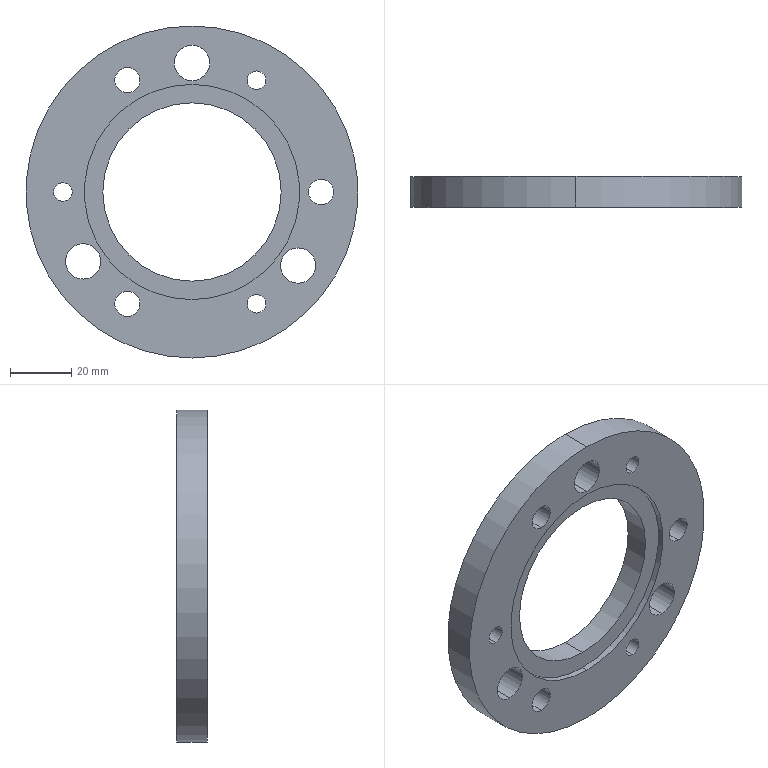Component | SolidWorks | Assembly4.1-1_116.1-1 | 1 solid | 27 faces | box 108 x 10 x 108 mm | volume 57227 mm3 | cylinder 24 | plane 3 | commonest cylinder face diameters 11.5 x6 8.2 x6 6 x6 70 x2 108 x2 58 x2
build123d program:
from build123d import *

# Parameters (mm, degrees)
SKETCH1_R                        = 54
SKETCH1_R_2                      = 29
BOSS_EXTRUDE1_DEPTH              = 10
CIRPATTERN1_COUNT                = 3
SKETCH4_R                        = 35
CUT_EXTRUDE1_DEPTH               = 2
F_8_2_8_2_DIAMETER_HOLE1_D       = 8.2
F_8_2_8_2_DIAMETER_HOLE1_DEPTH   = 15
F_8_2_8_2_DIAMETER_HOLE1_TIP     = 2.464
F_11_5_11_5_DIAMETER_HOLE1_D     = 11.5
F_11_5_11_5_DIAMETER_HOLE1_DEPTH = 15
F_11_5_11_5_DIAMETER_HOLE1_TIP   = 3.455


with BuildPart() as part:
    # Sketch1 → Boss-Extrude1 (new body)
    with BuildSketch(Plane.XY):
        Circle(SKETCH1_R)
        Circle(SKETCH1_R_2, mode=Mode.SUBTRACT)
    extrude(amount=BOSS_EXTRUDE1_DEPTH)

    # Sketch2 → 6.0 _6_ Diameter Hole1 (revolve, cut)
    with BuildSketch(Plane(origin=(0, 42, 10), x_dir=(0, -1, 0), z_dir=(1, 0, 0))):
        Polygon((0, 0), (0, 81.803), (3, 80), (3, 0), align=None)
    f_6_0_6_diameter_hole1 = revolve(axis=Axis((0, 42, 16.35), (0, 0, -1)), mode=Mode.SUBTRACT)

    # CirPattern1: 6.0 _6_ Diameter Hole1 ×3 about axis
    cirpattern1_axis = Axis((0, 0, 0), (0, 0, 1))
    for i in range(1, CIRPATTERN1_COUNT):
        add(f_6_0_6_diameter_hole1.rotate(cirpattern1_axis, i * 360 / CIRPATTERN1_COUNT), mode=Mode.SUBTRACT)

    # Sketch4 → Cut-Extrude1 (cut)
    with BuildSketch(Plane.XY.offset(10)):
        Circle(SKETCH4_R)
    extrude(amount=-CUT_EXTRUDE1_DEPTH, mode=Mode.SUBTRACT)

    # 8.2 _8.2_ Diameter Hole1
    with Locations(Plane.XY.offset(10)):
        with Locations((-36.373, 21), (36.373, 21), (0, -42)):
            Hole(F_8_2_8_2_DIAMETER_HOLE1_D / 2, depth=F_8_2_8_2_DIAMETER_HOLE1_DEPTH)
            with Locations((0, 0, -(F_8_2_8_2_DIAMETER_HOLE1_DEPTH + F_8_2_8_2_DIAMETER_HOLE1_TIP / 2))):  # 118° drill point
                Cone(0, F_8_2_8_2_DIAMETER_HOLE1_D / 2, F_8_2_8_2_DIAMETER_HOLE1_TIP, mode=Mode.SUBTRACT)

    # 11.5 _11.5_ Diameter Hole1
    with Locations(Plane.XY.offset(10)):
        with Locations((42, 0), (-23.935, -34.513), (-22.579, 35.415)):
            Hole(F_11_5_11_5_DIAMETER_HOLE1_D / 2, depth=F_11_5_11_5_DIAMETER_HOLE1_DEPTH)
            with Locations((0, 0, -(F_11_5_11_5_DIAMETER_HOLE1_DEPTH + F_11_5_11_5_DIAMETER_HOLE1_TIP / 2))):  # 118° drill point
                Cone(0, F_11_5_11_5_DIAMETER_HOLE1_D / 2, F_11_5_11_5_DIAMETER_HOLE1_TIP, mode=Mode.SUBTRACT)


solid = part.part

# Placed as in the assembly
solid = solid.moved(Location((0, -21.5, -0.4), (90, 0, 90)))
STEP:
#1=CARTESIAN_POINT('',(-0.,-0.8465,1.411));
#2=VERTEX_POINT('',#1);
#3=CARTESIAN_POINT('',(-0.,-0.8465,1.864));
#4=VERTEX_POINT('',#3);
#5=CARTESIAN_POINT('',(-0.,-0.8465,1.638));
#6=DIRECTION('',(-0.,-1.,0.));
#7=DIRECTION('',(-0.,0.,1.));
#8=AXIS2_PLACEMENT_3D('',#5,#6,#7);
#9=CIRCLE('',#8,0.2264);
#10=EDGE_CURVE('',#2,#4,#9,.T.);
#11=ORIENTED_EDGE('',*,*,#10,.F.);
#12=CARTESIAN_POINT('',(-0.,-1.24,1.411));
#13=VERTEX_POINT('',#12);
#14=CARTESIAN_POINT('',(-0.,-1.24,1.411));
#15=DIRECTION('',(-0.,-1.,0.));
#16=VECTOR('',#15,39.37);
#17=LINE('',#14,#16);
#18=EDGE_CURVE('',#2,#13,#17,.T.);
#19=ORIENTED_EDGE('',*,*,#18,.T.);
#20=CARTESIAN_POINT('',(-0.,-1.24,1.864));
#21=VERTEX_POINT('',#20);
#22=CARTESIAN_POINT('',(-0.,-1.24,1.638));
#23=DIRECTION('',(-0.,-1.,0.));
#24=DIRECTION('',(-0.,0.,1.));
#25=AXIS2_PLACEMENT_3D('',#22,#23,#24);
#26=CIRCLE('',#25,0.2264);
#27=EDGE_CURVE('',#13,#21,#26,.T.);
#28=ORIENTED_EDGE('',*,*,#27,.T.);
#29=CARTESIAN_POINT('',(-0.,-1.24,1.864));
#30=DIRECTION('',(-0.,-1.,0.));
#31=VECTOR('',#30,39.37);
#32=LINE('',#29,#31);
#33=EDGE_CURVE('',#4,#21,#32,.T.);
#34=ORIENTED_EDGE('',*,*,#33,.F.);
#35=EDGE_LOOP('',(#11,#19,#28,#34));
#36=FACE_OUTER_BOUND('',#35,.T.);
#37=CARTESIAN_POINT('',(-0.,-1.24,1.638));
#38=DIRECTION('',(-0.,-1.,0.));
#39=DIRECTION('',(-0.,0.,1.));
#40=AXIS2_PLACEMENT_3D('',#37,#38,#39);
#41=CYLINDRICAL_SURFACE('',#40,0.2264);
#42=ADVANCED_FACE('',(#36),#41,.F.);
#43=CARTESIAN_POINT('',(1.359,-0.8465,-1.184));
#44=VERTEX_POINT('',#43);
#45=CARTESIAN_POINT('',(1.359,-0.8465,-0.7317));
#46=VERTEX_POINT('',#45);
#47=CARTESIAN_POINT('',(1.359,-0.8465,-0.9581));
#48=DIRECTION('',(-0.,-1.,0.));
#49=DIRECTION('',(-0.,0.,1.));
#50=AXIS2_PLACEMENT_3D('',#47,#48,#49);
#51=CIRCLE('',#50,0.2264);
#52=EDGE_CURVE('',#44,#46,#51,.T.);
#53=ORIENTED_EDGE('',*,*,#52,.F.);
#54=CARTESIAN_POINT('',(1.359,-1.24,-1.184));
#55=VERTEX_POINT('',#54);
#56=CARTESIAN_POINT('',(1.359,-1.24,-1.184));
#57=DIRECTION('',(-0.,-1.,0.));
#58=VECTOR('',#57,39.37);
#59=LINE('',#56,#58);
#60=EDGE_CURVE('',#44,#55,#59,.T.);
#61=ORIENTED_EDGE('',*,*,#60,.T.);
#62=CARTESIAN_POINT('',(1.359,-1.24,-0.7317));
#63=VERTEX_POINT('',#62);
#64=CARTESIAN_POINT('',(1.359,-1.24,-0.9581));
#65=DIRECTION('',(-0.,-1.,0.));
#66=DIRECTION('',(-0.,0.,1.));
#67=AXIS2_PLACEMENT_3D('',#64,#65,#66);
#68=CIRCLE('',#67,0.2264);
#69=EDGE_CURVE('',#55,#63,#68,.T.);
#70=ORIENTED_EDGE('',*,*,#69,.T.);
#71=CARTESIAN_POINT('',(1.359,-1.24,-0.7317));
#72=DIRECTION('',(-0.,-1.,0.));
#73=VECTOR('',#72,39.37);
#74=LINE('',#71,#73);
#75=EDGE_CURVE('',#46,#63,#74,.T.);
#76=ORIENTED_EDGE('',*,*,#75,.F.);
#77=EDGE_LOOP('',(#53,#61,#70,#76));
#78=FACE_OUTER_BOUND('',#77,.T.);
#79=CARTESIAN_POINT('',(1.359,-1.24,-0.9581));
#80=DIRECTION('',(-0.,-1.,0.));
#81=DIRECTION('',(-0.,0.,1.));
#82=AXIS2_PLACEMENT_3D('',#79,#80,#81);
#83=CYLINDRICAL_SURFACE('',#82,0.2264);
#84=ADVANCED_FACE('',(#78),#83,.F.);
#85=CARTESIAN_POINT('',(-1.394,-0.8465,-1.131));
#86=VERTEX_POINT('',#85);
#87=CARTESIAN_POINT('',(-1.394,-0.8465,-0.6783));
#88=VERTEX_POINT('',#87);
#89=CARTESIAN_POINT('',(-1.394,-0.8465,-0.9047));
#90=DIRECTION('',(-0.,-1.,0.));
#91=DIRECTION('',(-0.,0.,1.));
#92=AXIS2_PLACEMENT_3D('',#89,#90,#91);
#93=CIRCLE('',#92,0.2264);
#94=EDGE_CURVE('',#86,#88,#93,.T.);
#95=ORIENTED_EDGE('',*,*,#94,.F.);
#96=CARTESIAN_POINT('',(-1.394,-1.24,-1.131));
#97=VERTEX_POINT('',#96);
#98=CARTESIAN_POINT('',(-1.394,-1.24,-1.131));
#99=DIRECTION('',(-0.,-1.,0.));
#100=VECTOR('',#99,39.37);
#101=LINE('',#98,#100);
#102=EDGE_CURVE('',#86,#97,#101,.T.);
#103=ORIENTED_EDGE('',*,*,#102,.T.);
#104=CARTESIAN_POINT('',(-1.394,-1.24,-0.6783));
#105=VERTEX_POINT('',#104);
#106=CARTESIAN_POINT('',(-1.394,-1.24,-0.9047));
#107=DIRECTION('',(-0.,-1.,0.));
#108=DIRECTION('',(-0.,0.,1.));
#109=AXIS2_PLACEMENT_3D('',#106,#107,#108);
#110=CIRCLE('',#109,0.2264);
#111=EDGE_CURVE('',#97,#105,#110,.T.);
#112=ORIENTED_EDGE('',*,*,#111,.T.);
#113=CARTESIAN_POINT('',(-1.394,-1.24,-0.6783));
#114=DIRECTION('',(-0.,-1.,0.));
#115=VECTOR('',#114,39.37);
#116=LINE('',#113,#115);
#117=EDGE_CURVE('',#88,#105,#116,.T.);
#118=ORIENTED_EDGE('',*,*,#117,.F.);
#119=EDGE_LOOP('',(#95,#103,#112,#118));
#120=FACE_OUTER_BOUND('',#119,.T.);
#121=CARTESIAN_POINT('',(-1.394,-1.24,-0.9047));
#122=DIRECTION('',(-0.,-1.,0.));
#123=DIRECTION('',(-0.,0.,1.));
#124=AXIS2_PLACEMENT_3D('',#121,#122,#123);
#125=CYLINDRICAL_SURFACE('',#124,0.2264);
#126=ADVANCED_FACE('',(#120),#125,.F.);
#127=CARTESIAN_POINT('',(-0.8268,-0.8465,-1.609));
#128=VERTEX_POINT('',#127);
#129=CARTESIAN_POINT('',(-0.8268,-0.8465,-1.286));
#130=VERTEX_POINT('',#129);
#131=CARTESIAN_POINT('',(-0.8268,-0.8465,-1.448));
#132=DIRECTION('',(-0.,-1.,0.));
#133=DIRECTION('',(-0.,0.,1.));
#134=AXIS2_PLACEMENT_3D('',#131,#132,#133);
#135=CIRCLE('',#134,0.1614);
#136=EDGE_CURVE('',#128,#130,#135,.T.);
#137=ORIENTED_EDGE('',*,*,#136,.F.);
#138=CARTESIAN_POINT('',(-0.8268,-1.24,-1.609));
#139=VERTEX_POINT('',#138);
#140=CARTESIAN_POINT('',(-0.8268,-1.24,-1.609));
#141=DIRECTION('',(-0.,-1.,0.));
#142=VECTOR('',#141,39.37);
#143=LINE('',#140,#142);
#144=EDGE_CURVE('',#128,#139,#143,.T.);
#145=ORIENTED_EDGE('',*,*,#144,.T.);
#146=CARTESIAN_POINT('',(-0.8268,-1.24,-1.286));
#147=VERTEX_POINT('',#146);
#148=CARTESIAN_POINT('',(-0.8268,-1.24,-1.448));
#149=DIRECTION('',(-0.,-1.,0.));
#150=DIRECTION('',(-0.,0.,1.));
#151=AXIS2_PLACEMENT_3D('',#148,#149,#150);
#152=CIRCLE('',#151,0.1614);
#153=EDGE_CURVE('',#139,#147,#152,.T.);
#154=ORIENTED_EDGE('',*,*,#153,.T.);
#155=CARTESIAN_POINT('',(-0.8268,-1.24,-1.286));
#156=DIRECTION('',(-0.,-1.,0.));
#157=VECTOR('',#156,39.37);
#158=LINE('',#155,#157);
#159=EDGE_CURVE('',#130,#147,#158,.T.);
#160=ORIENTED_EDGE('',*,*,#159,.F.);
#161=EDGE_LOOP('',(#137,#145,#154,#160));
#162=FACE_OUTER_BOUND('',#161,.T.);
#163=CARTESIAN_POINT('',(-0.8268,-1.24,-1.448));
#164=DIRECTION('',(-0.,-1.,0.));
#165=DIRECTION('',(-0.,0.,1.));
#166=AXIS2_PLACEMENT_3D('',#163,#164,#165);
#167=CYLINDRICAL_SURFACE('',#166,0.1614);
#168=ADVANCED_FACE('',(#162),#167,.F.);
#169=CARTESIAN_POINT('',(-0.8268,-0.8465,1.255));
#170=VERTEX_POINT('',#169);
#171=CARTESIAN_POINT('',(-0.8268,-0.8465,1.578));
#172=VERTEX_POINT('',#171);
#173=CARTESIAN_POINT('',(-0.8268,-0.8465,1.416));
#174=DIRECTION('',(-0.,-1.,0.));
#175=DIRECTION('',(-0.,0.,1.));
#176=AXIS2_PLACEMENT_3D('',#173,#174,#175);
#177=CIRCLE('',#176,0.1614);
#178=EDGE_CURVE('',#170,#172,#177,.T.);
#179=ORIENTED_EDGE('',*,*,#178,.F.);
#180=CARTESIAN_POINT('',(-0.8268,-1.24,1.255));
#181=VERTEX_POINT('',#180);
#182=CARTESIAN_POINT('',(-0.8268,-1.24,1.255));
#183=DIRECTION('',(-0.,-1.,0.));
#184=VECTOR('',#183,39.37);
#185=LINE('',#182,#184);
#186=EDGE_CURVE('',#170,#181,#185,.T.);
#187=ORIENTED_EDGE('',*,*,#186,.T.);
#188=CARTESIAN_POINT('',(-0.8268,-1.24,1.578));
#189=VERTEX_POINT('',#188);
#190=CARTESIAN_POINT('',(-0.8268,-1.24,1.416));
#191=DIRECTION('',(-0.,-1.,0.));
#192=DIRECTION('',(-0.,0.,1.));
#193=AXIS2_PLACEMENT_3D('',#190,#191,#192);
#194=CIRCLE('',#193,0.1614);
#195=EDGE_CURVE('',#181,#189,#194,.T.);
#196=ORIENTED_EDGE('',*,*,#195,.T.);
#197=CARTESIAN_POINT('',(-0.8268,-1.24,1.578));
#198=DIRECTION('',(-0.,-1.,0.));
#199=VECTOR('',#198,39.37);
#200=LINE('',#197,#199);
#201=EDGE_CURVE('',#172,#189,#200,.T.);
#202=ORIENTED_EDGE('',*,*,#201,.F.);
#203=EDGE_LOOP('',(#179,#187,#196,#202));
#204=FACE_OUTER_BOUND('',#203,.T.);
#205=CARTESIAN_POINT('',(-0.8268,-1.24,1.416));
#206=DIRECTION('',(-0.,-1.,0.));
#207=DIRECTION('',(-0.,0.,1.));
#208=AXIS2_PLACEMENT_3D('',#205,#206,#207);
#209=CYLINDRICAL_SURFACE('',#208,0.1614);
#210=ADVANCED_FACE('',(#204),#209,.F.);
#211=CARTESIAN_POINT('',(1.654,-0.8465,-0.1772));
#212=VERTEX_POINT('',#211);
#213=CARTESIAN_POINT('',(1.654,-0.8465,0.1457));
#214=VERTEX_POINT('',#213);
#215=CARTESIAN_POINT('',(1.654,-0.8465,-0.01575));
#216=DIRECTION('',(-0.,-1.,0.));
#217=DIRECTION('',(-0.,0.,1.));
#218=AXIS2_PLACEMENT_3D('',#215,#216,#217);
#219=CIRCLE('',#218,0.1614);
#220=EDGE_CURVE('',#212,#214,#219,.T.);
#221=ORIENTED_EDGE('',*,*,#220,.F.);
#222=CARTESIAN_POINT('',(1.654,-1.24,-0.1772));
#223=VERTEX_POINT('',#222);
#224=CARTESIAN_POINT('',(1.654,-1.24,-0.1772));
#225=DIRECTION('',(-0.,-1.,0.));
#226=VECTOR('',#225,39.37);
#227=LINE('',#224,#226);
#228=EDGE_CURVE('',#212,#223,#227,.T.);
#229=ORIENTED_EDGE('',*,*,#228,.T.);
#230=CARTESIAN_POINT('',(1.654,-1.24,0.1457));
#231=VERTEX_POINT('',#230);
#232=CARTESIAN_POINT('',(1.654,-1.24,-0.01575));
#233=DIRECTION('',(-0.,-1.,0.));
#234=DIRECTION('',(-0.,0.,1.));
#235=AXIS2_PLACEMENT_3D('',#232,#233,#234);
#236=CIRCLE('',#235,0.1614);
#237=EDGE_CURVE('',#223,#231,#236,.T.);
#238=ORIENTED_EDGE('',*,*,#237,.T.);
#239=CARTESIAN_POINT('',(1.654,-1.24,0.1457));
#240=DIRECTION('',(-0.,-1.,0.));
#241=VECTOR('',#240,39.37);
#242=LINE('',#239,#241);
#243=EDGE_CURVE('',#214,#231,#242,.T.);
#244=ORIENTED_EDGE('',*,*,#243,.F.);
#245=EDGE_LOOP('',(#221,#229,#238,#244));
#246=FACE_OUTER_BOUND('',#245,.T.);
#247=CARTESIAN_POINT('',(1.654,-1.24,-0.01575));
#248=DIRECTION('',(-0.,-1.,0.));
#249=DIRECTION('',(-0.,0.,1.));
#250=AXIS2_PLACEMENT_3D('',#247,#248,#249);
#251=CYLINDRICAL_SURFACE('',#250,0.1614);
#252=ADVANCED_FACE('',(#246),#251,.F.);
#253=CARTESIAN_POINT('',(0.,-1.161,-1.394));
#254=VERTEX_POINT('',#253);
#255=CARTESIAN_POINT('',(-0.,-1.161,1.362));
#256=VERTEX_POINT('',#255);
#257=CARTESIAN_POINT('',(-0.,-1.161,-0.01575));
#258=DIRECTION('',(-0.,-1.,0.));
#259=DIRECTION('',(-0.,0.,1.));
#260=AXIS2_PLACEMENT_3D('',#257,#258,#259);
#261=CIRCLE('',#260,1.378);
#262=EDGE_CURVE('',#254,#256,#261,.T.);
#263=ORIENTED_EDGE('',*,*,#262,.F.);
#264=CARTESIAN_POINT('',(0.,-1.24,-1.394));
#265=VERTEX_POINT('',#264);
#266=CARTESIAN_POINT('',(0.,-1.161,-1.394));
#267=DIRECTION('',(-0.,-1.,0.));
#268=VECTOR('',#267,39.37);
#269=LINE('',#266,#268);
#270=EDGE_CURVE('',#254,#265,#269,.T.);
#271=ORIENTED_EDGE('',*,*,#270,.T.);
#272=CARTESIAN_POINT('',(-0.,-1.24,1.362));
#273=VERTEX_POINT('',#272);
#274=CARTESIAN_POINT('',(-0.,-1.24,-0.01575));
#275=DIRECTION('',(-0.,-1.,0.));
#276=DIRECTION('',(-0.,0.,1.));
#277=AXIS2_PLACEMENT_3D('',#274,#275,#276);
#278=CIRCLE('',#277,1.378);
#279=EDGE_CURVE('',#265,#273,#278,.T.);
#280=ORIENTED_EDGE('',*,*,#279,.T.);
#281=CARTESIAN_POINT('',(-0.,-1.161,1.362));
#282=DIRECTION('',(-0.,-1.,0.));
#283=VECTOR('',#282,39.37);
#284=LINE('',#281,#283);
#285=EDGE_CURVE('',#256,#273,#284,.T.);
#286=ORIENTED_EDGE('',*,*,#285,.F.);
#287=EDGE_LOOP('',(#263,#271,#280,#286));
#288=FACE_OUTER_BOUND('',#287,.T.);
#289=CARTESIAN_POINT('',(-0.,-1.161,-0.01575));
#290=DIRECTION('',(-0.,-1.,0.));
#291=DIRECTION('',(-0.,0.,1.));
#292=AXIS2_PLACEMENT_3D('',#289,#290,#291);
#293=CYLINDRICAL_SURFACE('',#292,1.378);
#294=ADVANCED_FACE('',(#288),#293,.F.);
#295=CARTESIAN_POINT('',(0.8268,-0.8465,-1.566));
#296=VERTEX_POINT('',#295);
#297=CARTESIAN_POINT('',(0.8268,-0.8465,-1.33));
#298=VERTEX_POINT('',#297);
#299=CARTESIAN_POINT('',(0.8268,-0.8465,-1.448));
#300=DIRECTION('',(-0.,-1.,0.));
#301=DIRECTION('',(-0.,0.,1.));
#302=AXIS2_PLACEMENT_3D('',#299,#300,#301);
#303=CIRCLE('',#302,0.1181);
#304=EDGE_CURVE('',#296,#298,#303,.T.);
#305=ORIENTED_EDGE('',*,*,#304,.F.);
#306=CARTESIAN_POINT('',(0.8268,-1.24,-1.566));
#307=VERTEX_POINT('',#306);
#308=CARTESIAN_POINT('',(0.8268,-1.24,-1.566));
#309=DIRECTION('',(-0.,-1.,0.));
#310=VECTOR('',#309,39.37);
#311=LINE('',#308,#310);
#312=EDGE_CURVE('',#296,#307,#311,.T.);
#313=ORIENTED_EDGE('',*,*,#312,.T.);
#314=CARTESIAN_POINT('',(0.8268,-1.24,-1.33));
#315=VERTEX_POINT('',#314);
#316=CARTESIAN_POINT('',(0.8268,-1.24,-1.448));
#317=DIRECTION('',(-0.,-1.,0.));
#318=DIRECTION('',(-0.,0.,1.));
#319=AXIS2_PLACEMENT_3D('',#316,#317,#318);
#320=CIRCLE('',#319,0.1181);
#321=EDGE_CURVE('',#307,#315,#320,.T.);
#322=ORIENTED_EDGE('',*,*,#321,.T.);
#323=CARTESIAN_POINT('',(0.8268,-1.24,-1.33));
#324=DIRECTION('',(-0.,-1.,0.));
#325=VECTOR('',#324,39.37);
#326=LINE('',#323,#325);
#327=EDGE_CURVE('',#298,#315,#326,.T.);
#328=ORIENTED_EDGE('',*,*,#327,.F.);
#329=EDGE_LOOP('',(#305,#313,#322,#328));
#330=FACE_OUTER_BOUND('',#329,.T.);
#331=CARTESIAN_POINT('',(0.8268,-1.24,-1.448));
#332=DIRECTION('',(-0.,-1.,0.));
#333=DIRECTION('',(-0.,0.,1.));
#334=AXIS2_PLACEMENT_3D('',#331,#332,#333);
#335=CYLINDRICAL_SURFACE('',#334,0.1181);
#336=ADVANCED_FACE('',(#330),#335,.F.);
#337=CARTESIAN_POINT('',(0.8268,-0.8465,1.298));
#338=VERTEX_POINT('',#337);
#339=CARTESIAN_POINT('',(0.8268,-0.8465,1.534));
#340=VERTEX_POINT('',#339);
#341=CARTESIAN_POINT('',(0.8268,-0.8465,1.416));
#342=DIRECTION('',(-0.,-1.,0.));
#343=DIRECTION('',(-0.,0.,1.));
#344=AXIS2_PLACEMENT_3D('',#341,#342,#343);
#345=CIRCLE('',#344,0.1181);
#346=EDGE_CURVE('',#338,#340,#345,.T.);
#347=ORIENTED_EDGE('',*,*,#346,.F.);
#348=CARTESIAN_POINT('',(0.8268,-1.24,1.298));
#349=VERTEX_POINT('',#348);
#350=CARTESIAN_POINT('',(0.8268,-1.24,1.298));
#351=DIRECTION('',(-0.,-1.,0.));
#352=VECTOR('',#351,39.37);
#353=LINE('',#350,#352);
#354=EDGE_CURVE('',#338,#349,#353,.T.);
#355=ORIENTED_EDGE('',*,*,#354,.T.);
#356=CARTESIAN_POINT('',(0.8268,-1.24,1.534));
#357=VERTEX_POINT('',#356);
#358=CARTESIAN_POINT('',(0.8268,-1.24,1.416));
#359=DIRECTION('',(-0.,-1.,0.));
#360=DIRECTION('',(-0.,0.,1.));
#361=AXIS2_PLACEMENT_3D('',#358,#359,#360);
#362=CIRCLE('',#361,0.1181);
#363=EDGE_CURVE('',#349,#357,#362,.T.);
#364=ORIENTED_EDGE('',*,*,#363,.T.);
#365=CARTESIAN_POINT('',(0.8268,-1.24,1.534));
#366=DIRECTION('',(-0.,-1.,0.));
#367=VECTOR('',#366,39.37);
#368=LINE('',#365,#367);
#369=EDGE_CURVE('',#340,#357,#368,.T.);
#370=ORIENTED_EDGE('',*,*,#369,.F.);
#371=EDGE_LOOP('',(#347,#355,#364,#370));
#372=FACE_OUTER_BOUND('',#371,.T.);
#373=CARTESIAN_POINT('',(0.8268,-1.24,1.416));
#374=DIRECTION('',(-0.,-1.,0.));
#375=DIRECTION('',(-0.,0.,1.));
#376=AXIS2_PLACEMENT_3D('',#373,#374,#375);
#377=CYLINDRICAL_SURFACE('',#376,0.1181);
#378=ADVANCED_FACE('',(#372),#377,.F.);
#379=CARTESIAN_POINT('',(-1.654,-0.8465,-0.1339));
#380=VERTEX_POINT('',#379);
#381=CARTESIAN_POINT('',(-1.654,-0.8465,0.1024));
#382=VERTEX_POINT('',#381);
#383=CARTESIAN_POINT('',(-1.654,-0.8465,-0.01575));
#384=DIRECTION('',(-0.,-1.,0.));
#385=DIRECTION('',(-0.,0.,1.));
#386=AXIS2_PLACEMENT_3D('',#383,#384,#385);
#387=CIRCLE('',#386,0.1181);
#388=EDGE_CURVE('',#380,#382,#387,.T.);
#389=ORIENTED_EDGE('',*,*,#388,.F.);
#390=CARTESIAN_POINT('',(-1.654,-1.24,-0.1339));
#391=VERTEX_POINT('',#390);
#392=CARTESIAN_POINT('',(-1.654,-1.24,-0.1339));
#393=DIRECTION('',(-0.,-1.,0.));
#394=VECTOR('',#393,39.37);
#395=LINE('',#392,#394);
#396=EDGE_CURVE('',#380,#391,#395,.T.);
#397=ORIENTED_EDGE('',*,*,#396,.T.);
#398=CARTESIAN_POINT('',(-1.654,-1.24,0.1024));
#399=VERTEX_POINT('',#398);
#400=CARTESIAN_POINT('',(-1.654,-1.24,-0.01575));
#401=DIRECTION('',(-0.,-1.,0.));
#402=DIRECTION('',(-0.,0.,1.));
#403=AXIS2_PLACEMENT_3D('',#400,#401,#402);
#404=CIRCLE('',#403,0.1181);
#405=EDGE_CURVE('',#391,#399,#404,.T.);
#406=ORIENTED_EDGE('',*,*,#405,.T.);
#407=CARTESIAN_POINT('',(-1.654,-1.24,0.1024));
#408=DIRECTION('',(-0.,-1.,0.));
#409=VECTOR('',#408,39.37);
#410=LINE('',#407,#409);
#411=EDGE_CURVE('',#382,#399,#410,.T.);
#412=ORIENTED_EDGE('',*,*,#411,.F.);
#413=EDGE_LOOP('',(#389,#397,#406,#412));
#414=FACE_OUTER_BOUND('',#413,.T.);
#415=CARTESIAN_POINT('',(-1.654,-1.24,-0.01575));
#416=DIRECTION('',(-0.,-1.,0.));
#417=DIRECTION('',(-0.,0.,1.));
#418=AXIS2_PLACEMENT_3D('',#415,#416,#417);
#419=CYLINDRICAL_SURFACE('',#418,0.1181);
#420=ADVANCED_FACE('',(#414),#419,.F.);
#421=CARTESIAN_POINT('',(-0.,-1.24,2.11));
#422=VERTEX_POINT('',#421);
#423=CARTESIAN_POINT('',(0.,-1.24,-2.142));
#424=VERTEX_POINT('',#423);
#425=CARTESIAN_POINT('',(-0.,-1.24,-0.01575));
#426=DIRECTION('',(-0.,-1.,0.));
#427=DIRECTION('',(-0.,0.,1.));
#428=AXIS2_PLACEMENT_3D('',#425,#426,#427);
#429=CIRCLE('',#428,2.126);
#430=EDGE_CURVE('',#422,#424,#429,.T.);
#431=ORIENTED_EDGE('',*,*,#430,.F.);
#432=CARTESIAN_POINT('',(-0.,-0.8465,2.11));
#433=VERTEX_POINT('',#432);
#434=CARTESIAN_POINT('',(-0.,-1.24,2.11));
#435=DIRECTION('',(0.,1.,-0.));
#436=VECTOR('',#435,39.37);
#437=LINE('',#434,#436);
#438=EDGE_CURVE('',#422,#433,#437,.T.);
#439=ORIENTED_EDGE('',*,*,#438,.T.);
#440=CARTESIAN_POINT('',(0.,-0.8465,-2.142));
#441=VERTEX_POINT('',#440);
#442=CARTESIAN_POINT('',(-0.,-0.8465,-0.01575));
#443=DIRECTION('',(-0.,-1.,0.));
#444=DIRECTION('',(-0.,0.,1.));
#445=AXIS2_PLACEMENT_3D('',#442,#443,#444);
#446=CIRCLE('',#445,2.126);
#447=EDGE_CURVE('',#433,#441,#446,.T.);
#448=ORIENTED_EDGE('',*,*,#447,.T.);
#449=CARTESIAN_POINT('',(0.,-1.24,-2.142));
#450=DIRECTION('',(0.,1.,-0.));
#451=VECTOR('',#450,39.37);
#452=LINE('',#449,#451);
#453=EDGE_CURVE('',#424,#441,#452,.T.);
#454=ORIENTED_EDGE('',*,*,#453,.F.);
#455=EDGE_LOOP('',(#431,#439,#448,#454));
#456=FACE_OUTER_BOUND('',#455,.T.);
#457=CARTESIAN_POINT('',(-0.,-1.24,-0.01575));
#458=DIRECTION('',(0.,1.,-0.));
#459=DIRECTION('',(0.,0.,-1.));
#460=AXIS2_PLACEMENT_3D('',#457,#458,#459);
#461=CYLINDRICAL_SURFACE('',#460,2.126);
#462=ADVANCED_FACE('',(#456),#461,.T.);
#463=CARTESIAN_POINT('',(0.,-1.161,-1.157));
#464=VERTEX_POINT('',#463);
#465=CARTESIAN_POINT('',(-0.,-1.161,1.126));
#466=VERTEX_POINT('',#465);
#467=CARTESIAN_POINT('',(-0.,-1.161,-0.01575));
#468=DIRECTION('',(-0.,-1.,0.));
#469=DIRECTION('',(-0.,0.,1.));
#470=AXIS2_PLACEMENT_3D('',#467,#468,#469);
#471=CIRCLE('',#470,1.142);
#472=EDGE_CURVE('',#464,#466,#471,.T.);
#473=ORIENTED_EDGE('',*,*,#472,.T.);
#474=CARTESIAN_POINT('',(-0.,-0.8465,1.126));
#475=VERTEX_POINT('',#474);
#476=CARTESIAN_POINT('',(-0.,-1.24,1.126));
#477=DIRECTION('',(0.,1.,-0.));
#478=VECTOR('',#477,39.37);
#479=LINE('',#476,#478);
#480=EDGE_CURVE('',#466,#475,#479,.T.);
#481=ORIENTED_EDGE('',*,*,#480,.T.);
#482=CARTESIAN_POINT('',(0.,-0.8465,-1.157));
#483=VERTEX_POINT('',#482);
#484=CARTESIAN_POINT('',(-0.,-0.8465,-0.01575));
#485=DIRECTION('',(-0.,-1.,0.));
#486=DIRECTION('',(-0.,0.,1.));
#487=AXIS2_PLACEMENT_3D('',#484,#485,#486);
#488=CIRCLE('',#487,1.142);
#489=EDGE_CURVE('',#483,#475,#488,.T.);
#490=ORIENTED_EDGE('',*,*,#489,.F.);
#491=CARTESIAN_POINT('',(0.,-1.24,-1.157));
#492=DIRECTION('',(0.,1.,-0.));
#493=VECTOR('',#492,39.37);
#494=LINE('',#491,#493);
#495=EDGE_CURVE('',#464,#483,#494,.T.);
#496=ORIENTED_EDGE('',*,*,#495,.F.);
#497=EDGE_LOOP('',(#473,#481,#490,#496));
#498=FACE_OUTER_BOUND('',#497,.T.);
#499=CARTESIAN_POINT('',(-0.,-1.24,-0.01575));
#500=DIRECTION('',(0.,1.,-0.));
#501=DIRECTION('',(0.,0.,-1.));
#502=AXIS2_PLACEMENT_3D('',#499,#500,#501);
#503=CYLINDRICAL_SURFACE('',#502,1.142);
#504=ADVANCED_FACE('',(#498),#503,.F.);
#505=ORIENTED_EDGE('',*,*,#480,.F.);
#506=CARTESIAN_POINT('',(-0.,-1.161,-0.01575));
#507=DIRECTION('',(-0.,-1.,0.));
#508=DIRECTION('',(-0.,0.,1.));
#509=AXIS2_PLACEMENT_3D('',#506,#507,#508);
#510=CIRCLE('',#509,1.142);
#511=EDGE_CURVE('',#466,#464,#510,.T.);
#512=ORIENTED_EDGE('',*,*,#511,.T.);
#513=ORIENTED_EDGE('',*,*,#495,.T.);
#514=CARTESIAN_POINT('',(-0.,-0.8465,-0.01575));
#515=DIRECTION('',(-0.,-1.,0.));
#516=DIRECTION('',(-0.,0.,1.));
#517=AXIS2_PLACEMENT_3D('',#514,#515,#516);
#518=CIRCLE('',#517,1.142);
#519=EDGE_CURVE('',#475,#483,#518,.T.);
#520=ORIENTED_EDGE('',*,*,#519,.F.);
#521=EDGE_LOOP('',(#505,#512,#513,#520));
#522=FACE_OUTER_BOUND('',#521,.T.);
#523=CARTESIAN_POINT('',(-0.,-1.24,-0.01575));
#524=DIRECTION('',(0.,1.,-0.));
#525=DIRECTION('',(0.,0.,-1.));
#526=AXIS2_PLACEMENT_3D('',#523,#524,#525);
#527=CYLINDRICAL_SURFACE('',#526,1.142);
#528=ADVANCED_FACE('',(#522),#527,.F.);
#529=CARTESIAN_POINT('',(-0.,-1.24,1.638));
#530=DIRECTION('',(-0.,-1.,0.));
#531=DIRECTION('',(-0.,0.,1.));
#532=AXIS2_PLACEMENT_3D('',#529,#530,#531);
#533=CIRCLE('',#532,0.2264);
#534=EDGE_CURVE('',#21,#13,#533,.T.);
#535=ORIENTED_EDGE('',*,*,#534,.F.);
#536=ORIENTED_EDGE('',*,*,#27,.F.);
#537=EDGE_LOOP('',(#535,#536));
#538=FACE_BOUND('',#537,.T.);
#539=CARTESIAN_POINT('',(1.359,-1.24,-0.9581));
#540=DIRECTION('',(-0.,-1.,0.));
#541=DIRECTION('',(-0.,0.,1.));
#542=AXIS2_PLACEMENT_3D('',#539,#540,#541);
#543=CIRCLE('',#542,0.2264);
#544=EDGE_CURVE('',#63,#55,#543,.T.);
#545=ORIENTED_EDGE('',*,*,#544,.F.);
#546=ORIENTED_EDGE('',*,*,#69,.F.);
#547=EDGE_LOOP('',(#545,#546));
#548=FACE_BOUND('',#547,.T.);
#549=CARTESIAN_POINT('',(-1.394,-1.24,-0.9047));
#550=DIRECTION('',(-0.,-1.,0.));
#551=DIRECTION('',(-0.,0.,1.));
#552=AXIS2_PLACEMENT_3D('',#549,#550,#551);
#553=CIRCLE('',#552,0.2264);
#554=EDGE_CURVE('',#105,#97,#553,.T.);
#555=ORIENTED_EDGE('',*,*,#554,.F.);
#556=ORIENTED_EDGE('',*,*,#111,.F.);
#557=EDGE_LOOP('',(#555,#556));
#558=FACE_BOUND('',#557,.T.);
#559=CARTESIAN_POINT('',(-0.8268,-1.24,-1.448));
#560=DIRECTION('',(-0.,-1.,0.));
#561=DIRECTION('',(-0.,0.,1.));
#562=AXIS2_PLACEMENT_3D('',#559,#560,#561);
#563=CIRCLE('',#562,0.1614);
#564=EDGE_CURVE('',#147,#139,#563,.T.);
#565=ORIENTED_EDGE('',*,*,#564,.F.);
#566=ORIENTED_EDGE('',*,*,#153,.F.);
#567=EDGE_LOOP('',(#565,#566));
#568=FACE_BOUND('',#567,.T.);
#569=CARTESIAN_POINT('',(-0.8268,-1.24,1.416));
#570=DIRECTION('',(-0.,-1.,0.));
#571=DIRECTION('',(-0.,0.,1.));
#572=AXIS2_PLACEMENT_3D('',#569,#570,#571);
#573=CIRCLE('',#572,0.1614);
#574=EDGE_CURVE('',#189,#181,#573,.T.);
#575=ORIENTED_EDGE('',*,*,#574,.F.);
#576=ORIENTED_EDGE('',*,*,#195,.F.);
#577=EDGE_LOOP('',(#575,#576));
#578=FACE_BOUND('',#577,.T.);
#579=CARTESIAN_POINT('',(1.654,-1.24,-0.01575));
#580=DIRECTION('',(-0.,-1.,0.));
#581=DIRECTION('',(-0.,0.,1.));
#582=AXIS2_PLACEMENT_3D('',#579,#580,#581);
#583=CIRCLE('',#582,0.1614);
#584=EDGE_CURVE('',#231,#223,#583,.T.);
#585=ORIENTED_EDGE('',*,*,#584,.F.);
#586=ORIENTED_EDGE('',*,*,#237,.F.);
#587=EDGE_LOOP('',(#585,#586));
#588=FACE_BOUND('',#587,.T.);
#589=CARTESIAN_POINT('',(-0.,-1.24,-0.01575));
#590=DIRECTION('',(-0.,-1.,0.));
#591=DIRECTION('',(-0.,0.,1.));
#592=AXIS2_PLACEMENT_3D('',#589,#590,#591);
#593=CIRCLE('',#592,1.378);
#594=EDGE_CURVE('',#273,#265,#593,.T.);
#595=ORIENTED_EDGE('',*,*,#594,.F.);
#596=ORIENTED_EDGE('',*,*,#279,.F.);
#597=EDGE_LOOP('',(#595,#596));
#598=FACE_BOUND('',#597,.T.);
#599=CARTESIAN_POINT('',(0.8268,-1.24,-1.448));
#600=DIRECTION('',(-0.,-1.,0.));
#601=DIRECTION('',(-0.,0.,1.));
#602=AXIS2_PLACEMENT_3D('',#599,#600,#601);
#603=CIRCLE('',#602,0.1181);
#604=EDGE_CURVE('',#315,#307,#603,.T.);
#605=ORIENTED_EDGE('',*,*,#604,.F.);
#606=ORIENTED_EDGE('',*,*,#321,.F.);
#607=EDGE_LOOP('',(#605,#606));
#608=FACE_BOUND('',#607,.T.);
#609=CARTESIAN_POINT('',(0.8268,-1.24,1.416));
#610=DIRECTION('',(-0.,-1.,0.));
#611=DIRECTION('',(-0.,0.,1.));
#612=AXIS2_PLACEMENT_3D('',#609,#610,#611);
#613=CIRCLE('',#612,0.1181);
#614=EDGE_CURVE('',#357,#349,#613,.T.);
#615=ORIENTED_EDGE('',*,*,#614,.F.);
#616=ORIENTED_EDGE('',*,*,#363,.F.);
#617=EDGE_LOOP('',(#615,#616));
#618=FACE_BOUND('',#617,.T.);
#619=CARTESIAN_POINT('',(-1.654,-1.24,-0.01575));
#620=DIRECTION('',(-0.,-1.,0.));
#621=DIRECTION('',(-0.,0.,1.));
#622=AXIS2_PLACEMENT_3D('',#619,#620,#621);
#623=CIRCLE('',#622,0.1181);
#624=EDGE_CURVE('',#399,#391,#623,.T.);
#625=ORIENTED_EDGE('',*,*,#624,.F.);
#626=ORIENTED_EDGE('',*,*,#405,.F.);
#627=EDGE_LOOP('',(#625,#626));
#628=FACE_BOUND('',#627,.T.);
#629=CARTESIAN_POINT('',(-0.,-1.24,-0.01575));
#630=DIRECTION('',(-0.,-1.,0.));
#631=DIRECTION('',(-0.,0.,1.));
#632=AXIS2_PLACEMENT_3D('',#629,#630,#631);
#633=CIRCLE('',#632,2.126);
#634=EDGE_CURVE('',#424,#422,#633,.T.);
#635=ORIENTED_EDGE('',*,*,#634,.T.);
#636=ORIENTED_EDGE('',*,*,#430,.T.);
#637=EDGE_LOOP('',(#635,#636));
#638=FACE_OUTER_BOUND('',#637,.T.);
#639=CARTESIAN_POINT('',(-0.,-1.24,-0.01575));
#640=DIRECTION('',(-0.,-1.,0.));
#641=DIRECTION('',(-0.,0.,1.));
#642=AXIS2_PLACEMENT_3D('',#639,#640,#641);
#643=PLANE('',#642);
#644=ADVANCED_FACE('',(#538,#548,#558,#568,#578,#588,#598,#608,#618,#628,#638),#643,.T.);
#645=CARTESIAN_POINT('',(-0.,-0.8465,1.638));
#646=DIRECTION('',(-0.,-1.,0.));
#647=DIRECTION('',(-0.,0.,1.));
#648=AXIS2_PLACEMENT_3D('',#645,#646,#647);
#649=CIRCLE('',#648,0.2264);
#650=EDGE_CURVE('',#4,#2,#649,.T.);
#651=ORIENTED_EDGE('',*,*,#650,.T.);
#652=ORIENTED_EDGE('',*,*,#10,.T.);
#653=EDGE_LOOP('',(#651,#652));
#654=FACE_BOUND('',#653,.T.);
#655=CARTESIAN_POINT('',(1.359,-0.8465,-0.9581));
#656=DIRECTION('',(-0.,-1.,0.));
#657=DIRECTION('',(-0.,0.,1.));
#658=AXIS2_PLACEMENT_3D('',#655,#656,#657);
#659=CIRCLE('',#658,0.2264);
#660=EDGE_CURVE('',#46,#44,#659,.T.);
#661=ORIENTED_EDGE('',*,*,#660,.T.);
#662=ORIENTED_EDGE('',*,*,#52,.T.);
#663=EDGE_LOOP('',(#661,#662));
#664=FACE_BOUND('',#663,.T.);
#665=CARTESIAN_POINT('',(-1.394,-0.8465,-0.9047));
#666=DIRECTION('',(-0.,-1.,0.));
#667=DIRECTION('',(-0.,0.,1.));
#668=AXIS2_PLACEMENT_3D('',#665,#666,#667);
#669=CIRCLE('',#668,0.2264);
#670=EDGE_CURVE('',#88,#86,#669,.T.);
#671=ORIENTED_EDGE('',*,*,#670,.T.);
#672=ORIENTED_EDGE('',*,*,#94,.T.);
#673=EDGE_LOOP('',(#671,#672));
#674=FACE_BOUND('',#673,.T.);
#675=CARTESIAN_POINT('',(-0.8268,-0.8465,-1.448));
#676=DIRECTION('',(-0.,-1.,0.));
#677=DIRECTION('',(-0.,0.,1.));
#678=AXIS2_PLACEMENT_3D('',#675,#676,#677);
#679=CIRCLE('',#678,0.1614);
#680=EDGE_CURVE('',#130,#128,#679,.T.);
#681=ORIENTED_EDGE('',*,*,#680,.T.);
#682=ORIENTED_EDGE('',*,*,#136,.T.);
#683=EDGE_LOOP('',(#681,#682));
#684=FACE_BOUND('',#683,.T.);
#685=CARTESIAN_POINT('',(-0.8268,-0.8465,1.416));
#686=DIRECTION('',(-0.,-1.,0.));
#687=DIRECTION('',(-0.,0.,1.));
#688=AXIS2_PLACEMENT_3D('',#685,#686,#687);
#689=CIRCLE('',#688,0.1614);
#690=EDGE_CURVE('',#172,#170,#689,.T.);
#691=ORIENTED_EDGE('',*,*,#690,.T.);
#692=ORIENTED_EDGE('',*,*,#178,.T.);
#693=EDGE_LOOP('',(#691,#692));
#694=FACE_BOUND('',#693,.T.);
#695=CARTESIAN_POINT('',(1.654,-0.8465,-0.01575));
#696=DIRECTION('',(-0.,-1.,0.));
#697=DIRECTION('',(-0.,0.,1.));
#698=AXIS2_PLACEMENT_3D('',#695,#696,#697);
#699=CIRCLE('',#698,0.1614);
#700=EDGE_CURVE('',#214,#212,#699,.T.);
#701=ORIENTED_EDGE('',*,*,#700,.T.);
#702=ORIENTED_EDGE('',*,*,#220,.T.);
#703=EDGE_LOOP('',(#701,#702));
#704=FACE_BOUND('',#703,.T.);
#705=CARTESIAN_POINT('',(0.8268,-0.8465,-1.448));
#706=DIRECTION('',(-0.,-1.,0.));
#707=DIRECTION('',(-0.,0.,1.));
#708=AXIS2_PLACEMENT_3D('',#705,#706,#707);
#709=CIRCLE('',#708,0.1181);
#710=EDGE_CURVE('',#298,#296,#709,.T.);
#711=ORIENTED_EDGE('',*,*,#710,.T.);
#712=ORIENTED_EDGE('',*,*,#304,.T.);
#713=EDGE_LOOP('',(#711,#712));
#714=FACE_BOUND('',#713,.T.);
#715=CARTESIAN_POINT('',(0.8268,-0.8465,1.416));
#716=DIRECTION('',(-0.,-1.,0.));
#717=DIRECTION('',(-0.,0.,1.));
#718=AXIS2_PLACEMENT_3D('',#715,#716,#717);
#719=CIRCLE('',#718,0.1181);
#720=EDGE_CURVE('',#340,#338,#719,.T.);
#721=ORIENTED_EDGE('',*,*,#720,.T.);
#722=ORIENTED_EDGE('',*,*,#346,.T.);
#723=EDGE_LOOP('',(#721,#722));
#724=FACE_BOUND('',#723,.T.);
#725=CARTESIAN_POINT('',(-1.654,-0.8465,-0.01575));
#726=DIRECTION('',(-0.,-1.,0.));
#727=DIRECTION('',(-0.,0.,1.));
#728=AXIS2_PLACEMENT_3D('',#725,#726,#727);
#729=CIRCLE('',#728,0.1181);
#730=EDGE_CURVE('',#382,#380,#729,.T.);
#731=ORIENTED_EDGE('',*,*,#730,.T.);
#732=ORIENTED_EDGE('',*,*,#388,.T.);
#733=EDGE_LOOP('',(#731,#732));
#734=FACE_BOUND('',#733,.T.);
#735=CARTESIAN_POINT('',(-0.,-0.8465,-0.01575));
#736=DIRECTION('',(-0.,-1.,0.));
#737=DIRECTION('',(-0.,0.,1.));
#738=AXIS2_PLACEMENT_3D('',#735,#736,#737);
#739=CIRCLE('',#738,2.126);
#740=EDGE_CURVE('',#441,#433,#739,.T.);
#741=ORIENTED_EDGE('',*,*,#740,.F.);
#742=ORIENTED_EDGE('',*,*,#447,.F.);
#743=EDGE_LOOP('',(#741,#742));
#744=FACE_OUTER_BOUND('',#743,.T.);
#745=ORIENTED_EDGE('',*,*,#489,.T.);
#746=ORIENTED_EDGE('',*,*,#519,.T.);
#747=EDGE_LOOP('',(#745,#746));
#748=FACE_BOUND('',#747,.T.);
#749=CARTESIAN_POINT('',(-0.,-0.8465,-0.01575));
#750=DIRECTION('',(-0.,-1.,0.));
#751=DIRECTION('',(-0.,0.,1.));
#752=AXIS2_PLACEMENT_3D('',#749,#750,#751);
#753=PLANE('',#752);
#754=ADVANCED_FACE('',(#654,#664,#674,#684,#694,#704,#714,#724,#734,#744,#748),#753,.F.);
#755=ORIENTED_EDGE('',*,*,#438,.F.);
#756=ORIENTED_EDGE('',*,*,#634,.F.);
#757=ORIENTED_EDGE('',*,*,#453,.T.);
#758=ORIENTED_EDGE('',*,*,#740,.T.);
#759=EDGE_LOOP('',(#755,#756,#757,#758));
#760=FACE_OUTER_BOUND('',#759,.T.);
#761=CARTESIAN_POINT('',(-0.,-1.24,-0.01575));
#762=DIRECTION('',(0.,1.,-0.));
#763=DIRECTION('',(0.,0.,-1.));
#764=AXIS2_PLACEMENT_3D('',#761,#762,#763);
#765=CYLINDRICAL_SURFACE('',#764,2.126);
#766=ADVANCED_FACE('',(#760),#765,.T.);
#767=ORIENTED_EDGE('',*,*,#396,.F.);
#768=ORIENTED_EDGE('',*,*,#730,.F.);
#769=ORIENTED_EDGE('',*,*,#411,.T.);
#770=ORIENTED_EDGE('',*,*,#624,.T.);
#771=EDGE_LOOP('',(#767,#768,#769,#770));
#772=FACE_OUTER_BOUND('',#771,.T.);
#773=CARTESIAN_POINT('',(-1.654,-1.24,-0.01575));
#774=DIRECTION('',(-0.,-1.,0.));
#775=DIRECTION('',(-0.,0.,1.));
#776=AXIS2_PLACEMENT_3D('',#773,#774,#775);
#777=CYLINDRICAL_SURFACE('',#776,0.1181);
#778=ADVANCED_FACE('',(#772),#777,.F.);
#779=ORIENTED_EDGE('',*,*,#354,.F.);
#780=ORIENTED_EDGE('',*,*,#720,.F.);
#781=ORIENTED_EDGE('',*,*,#369,.T.);
#782=ORIENTED_EDGE('',*,*,#614,.T.);
#783=EDGE_LOOP('',(#779,#780,#781,#782));
#784=FACE_OUTER_BOUND('',#783,.T.);
#785=CARTESIAN_POINT('',(0.8268,-1.24,1.416));
#786=DIRECTION('',(-0.,-1.,0.));
#787=DIRECTION('',(-0.,0.,1.));
#788=AXIS2_PLACEMENT_3D('',#785,#786,#787);
#789=CYLINDRICAL_SURFACE('',#788,0.1181);
#790=ADVANCED_FACE('',(#784),#789,.F.);
#791=ORIENTED_EDGE('',*,*,#312,.F.);
#792=ORIENTED_EDGE('',*,*,#710,.F.);
#793=ORIENTED_EDGE('',*,*,#327,.T.);
#794=ORIENTED_EDGE('',*,*,#604,.T.);
#795=EDGE_LOOP('',(#791,#792,#793,#794));
#796=FACE_OUTER_BOUND('',#795,.T.);
#797=CARTESIAN_POINT('',(0.8268,-1.24,-1.448));
#798=DIRECTION('',(-0.,-1.,0.));
#799=DIRECTION('',(-0.,0.,1.));
#800=AXIS2_PLACEMENT_3D('',#797,#798,#799);
#801=CYLINDRICAL_SURFACE('',#800,0.1181);
#802=ADVANCED_FACE('',(#796),#801,.F.);
#803=ORIENTED_EDGE('',*,*,#270,.F.);
#804=CARTESIAN_POINT('',(-0.,-1.161,-0.01575));
#805=DIRECTION('',(-0.,-1.,0.));
#806=DIRECTION('',(-0.,0.,1.));
#807=AXIS2_PLACEMENT_3D('',#804,#805,#806);
#808=CIRCLE('',#807,1.378);
#809=EDGE_CURVE('',#256,#254,#808,.T.);
#810=ORIENTED_EDGE('',*,*,#809,.F.);
#811=ORIENTED_EDGE('',*,*,#285,.T.);
#812=ORIENTED_EDGE('',*,*,#594,.T.);
#813=EDGE_LOOP('',(#803,#810,#811,#812));
#814=FACE_OUTER_BOUND('',#813,.T.);
#815=CARTESIAN_POINT('',(-0.,-1.161,-0.01575));
#816=DIRECTION('',(-0.,-1.,0.));
#817=DIRECTION('',(-0.,0.,1.));
#818=AXIS2_PLACEMENT_3D('',#815,#816,#817);
#819=CYLINDRICAL_SURFACE('',#818,1.378);
#820=ADVANCED_FACE('',(#814),#819,.F.);
#821=ORIENTED_EDGE('',*,*,#472,.F.);
#822=ORIENTED_EDGE('',*,*,#511,.F.);
#823=EDGE_LOOP('',(#821,#822));
#824=FACE_BOUND('',#823,.T.);
#825=ORIENTED_EDGE('',*,*,#809,.T.);
#826=ORIENTED_EDGE('',*,*,#262,.T.);
#827=EDGE_LOOP('',(#825,#826));
#828=FACE_OUTER_BOUND('',#827,.T.);
#829=CARTESIAN_POINT('',(-0.,-1.161,-0.01575));
#830=DIRECTION('',(-0.,-1.,0.));
#831=DIRECTION('',(-0.,0.,1.));
#832=AXIS2_PLACEMENT_3D('',#829,#830,#831);
#833=PLANE('',#832);
#834=ADVANCED_FACE('',(#824,#828),#833,.T.);
#835=ORIENTED_EDGE('',*,*,#228,.F.);
#836=ORIENTED_EDGE('',*,*,#700,.F.);
#837=ORIENTED_EDGE('',*,*,#243,.T.);
#838=ORIENTED_EDGE('',*,*,#584,.T.);
#839=EDGE_LOOP('',(#835,#836,#837,#838));
#840=FACE_OUTER_BOUND('',#839,.T.);
#841=CARTESIAN_POINT('',(1.654,-1.24,-0.01575));
#842=DIRECTION('',(-0.,-1.,0.));
#843=DIRECTION('',(-0.,0.,1.));
#844=AXIS2_PLACEMENT_3D('',#841,#842,#843);
#845=CYLINDRICAL_SURFACE('',#844,0.1614);
#846=ADVANCED_FACE('',(#840),#845,.F.);
#847=ORIENTED_EDGE('',*,*,#186,.F.);
#848=ORIENTED_EDGE('',*,*,#690,.F.);
#849=ORIENTED_EDGE('',*,*,#201,.T.);
#850=ORIENTED_EDGE('',*,*,#574,.T.);
#851=EDGE_LOOP('',(#847,#848,#849,#850));
#852=FACE_OUTER_BOUND('',#851,.T.);
#853=CARTESIAN_POINT('',(-0.8268,-1.24,1.416));
#854=DIRECTION('',(-0.,-1.,0.));
#855=DIRECTION('',(-0.,0.,1.));
#856=AXIS2_PLACEMENT_3D('',#853,#854,#855);
#857=CYLINDRICAL_SURFACE('',#856,0.1614);
#858=ADVANCED_FACE('',(#852),#857,.F.);
#859=ORIENTED_EDGE('',*,*,#144,.F.);
#860=ORIENTED_EDGE('',*,*,#680,.F.);
#861=ORIENTED_EDGE('',*,*,#159,.T.);
#862=ORIENTED_EDGE('',*,*,#564,.T.);
#863=EDGE_LOOP('',(#859,#860,#861,#862));
#864=FACE_OUTER_BOUND('',#863,.T.);
#865=CARTESIAN_POINT('',(-0.8268,-1.24,-1.448));
#866=DIRECTION('',(-0.,-1.,0.));
#867=DIRECTION('',(-0.,0.,1.));
#868=AXIS2_PLACEMENT_3D('',#865,#866,#867);
#869=CYLINDRICAL_SURFACE('',#868,0.1614);
#870=ADVANCED_FACE('',(#864),#869,.F.);
#871=ORIENTED_EDGE('',*,*,#102,.F.);
#872=ORIENTED_EDGE('',*,*,#670,.F.);
#873=ORIENTED_EDGE('',*,*,#117,.T.);
#874=ORIENTED_EDGE('',*,*,#554,.T.);
#875=EDGE_LOOP('',(#871,#872,#873,#874));
#876=FACE_OUTER_BOUND('',#875,.T.);
#877=CARTESIAN_POINT('',(-1.394,-1.24,-0.9047));
#878=DIRECTION('',(-0.,-1.,0.));
#879=DIRECTION('',(-0.,0.,1.));
#880=AXIS2_PLACEMENT_3D('',#877,#878,#879);
#881=CYLINDRICAL_SURFACE('',#880,0.2264);
#882=ADVANCED_FACE('',(#876),#881,.F.);
#883=ORIENTED_EDGE('',*,*,#60,.F.);
#884=ORIENTED_EDGE('',*,*,#660,.F.);
#885=ORIENTED_EDGE('',*,*,#75,.T.);
#886=ORIENTED_EDGE('',*,*,#544,.T.);
#887=EDGE_LOOP('',(#883,#884,#885,#886));
#888=FACE_OUTER_BOUND('',#887,.T.);
#889=CARTESIAN_POINT('',(1.359,-1.24,-0.9581));
#890=DIRECTION('',(-0.,-1.,0.));
#891=DIRECTION('',(-0.,0.,1.));
#892=AXIS2_PLACEMENT_3D('',#889,#890,#891);
#893=CYLINDRICAL_SURFACE('',#892,0.2264);
#894=ADVANCED_FACE('',(#888),#893,.F.);
#895=ORIENTED_EDGE('',*,*,#18,.F.);
#896=ORIENTED_EDGE('',*,*,#650,.F.);
#897=ORIENTED_EDGE('',*,*,#33,.T.);
#898=ORIENTED_EDGE('',*,*,#534,.T.);
#899=EDGE_LOOP('',(#895,#896,#897,#898));
#900=FACE_OUTER_BOUND('',#899,.T.);
#901=CARTESIAN_POINT('',(-0.,-1.24,1.638));
#902=DIRECTION('',(-0.,-1.,0.));
#903=DIRECTION('',(-0.,0.,1.));
#904=AXIS2_PLACEMENT_3D('',#901,#902,#903);
#905=CYLINDRICAL_SURFACE('',#904,0.2264);
#906=ADVANCED_FACE('',(#900),#905,.F.);
#907=CLOSED_SHELL('',(#42,#84,#126,#168,#210,#252,#294,#336,#378,#420,#462,#504,#528,#644,#754,#766,#778,#790,#802,#820,#834,#846,#858,#870,#882,#894,#906));
#908=MANIFOLD_SOLID_BREP('',#907);
#909=CARTESIAN_POINT('',(0.,0.,0.));
#910=DIRECTION('',(0.,0.,1.));
#911=DIRECTION('',(1.,0.,0.));
#912=AXIS2_PLACEMENT_3D('',#909,#910,#911);
#913=(LENGTH_UNIT()NAMED_UNIT(*)SI_UNIT($,.METRE.));
#914=LENGTH_MEASURE_WITH_UNIT(LENGTH_MEASURE(0.0254),#913);
#915=DIMENSIONAL_EXPONENTS(1.,0.,0.,0.,0.,0.,0.);
#916=(CONVERSION_BASED_UNIT('',#914)LENGTH_UNIT()NAMED_UNIT(#915));
#917=UNCERTAINTY_MEASURE_WITH_UNIT(LENGTH_MEASURE(0.00001),#916,'','');
#918=(NAMED_UNIT(*)PLANE_ANGLE_UNIT()SI_UNIT($,.RADIAN.));
#919=(NAMED_UNIT(*)SI_UNIT($,.STERADIAN.)SOLID_ANGLE_UNIT());
#920=(GEOMETRIC_REPRESENTATION_CONTEXT(3)GLOBAL_UNCERTAINTY_ASSIGNED_CONTEXT((#917))GLOBAL_UNIT_ASSIGNED_CONTEXT((#916,#918,#919))REPRESENTATION_CONTEXT('',''));
#921=ADVANCED_BREP_SHAPE_REPRESENTATION('',(#908,#912),#920);
#922=COLOUR_RGB('',0.7922,0.8196,0.9333);
#923=FILL_AREA_STYLE_COLOUR('',#922);
#924=FILL_AREA_STYLE('',(#923));
#925=SURFACE_STYLE_FILL_AREA(#924);
#926=SURFACE_SIDE_STYLE('',(#925));
#927=SURFACE_STYLE_USAGE(.BOTH.,#926);
#928=PRESENTATION_STYLE_ASSIGNMENT((#927));
#929=STYLED_ITEM('',(#928),#908);
#930=(LENGTH_UNIT()NAMED_UNIT(*)SI_UNIT($,.METRE.));
#931=LENGTH_MEASURE_WITH_UNIT(LENGTH_MEASURE(0.0254),#930);
#932=DIMENSIONAL_EXPONENTS(1.,0.,0.,0.,0.,0.,0.);
#933=(CONVERSION_BASED_UNIT('',#931)LENGTH_UNIT()NAMED_UNIT(#932));
#934=UNCERTAINTY_MEASURE_WITH_UNIT(LENGTH_MEASURE(0.00001),#933,'','');
#935=(NAMED_UNIT(*)PLANE_ANGLE_UNIT()SI_UNIT($,.RADIAN.));
#936=(NAMED_UNIT(*)SI_UNIT($,.STERADIAN.)SOLID_ANGLE_UNIT());
#937=(GEOMETRIC_REPRESENTATION_CONTEXT(3)GLOBAL_UNCERTAINTY_ASSIGNED_CONTEXT((#934))GLOBAL_UNIT_ASSIGNED_CONTEXT((#933,#935,#936))REPRESENTATION_CONTEXT('',''));
#938=MECHANICAL_DESIGN_GEOMETRIC_PRESENTATION_REPRESENTATION('',(#929),#937);
#939=PRESENTATION_LAYER_ASSIGNMENT('','',(#929));